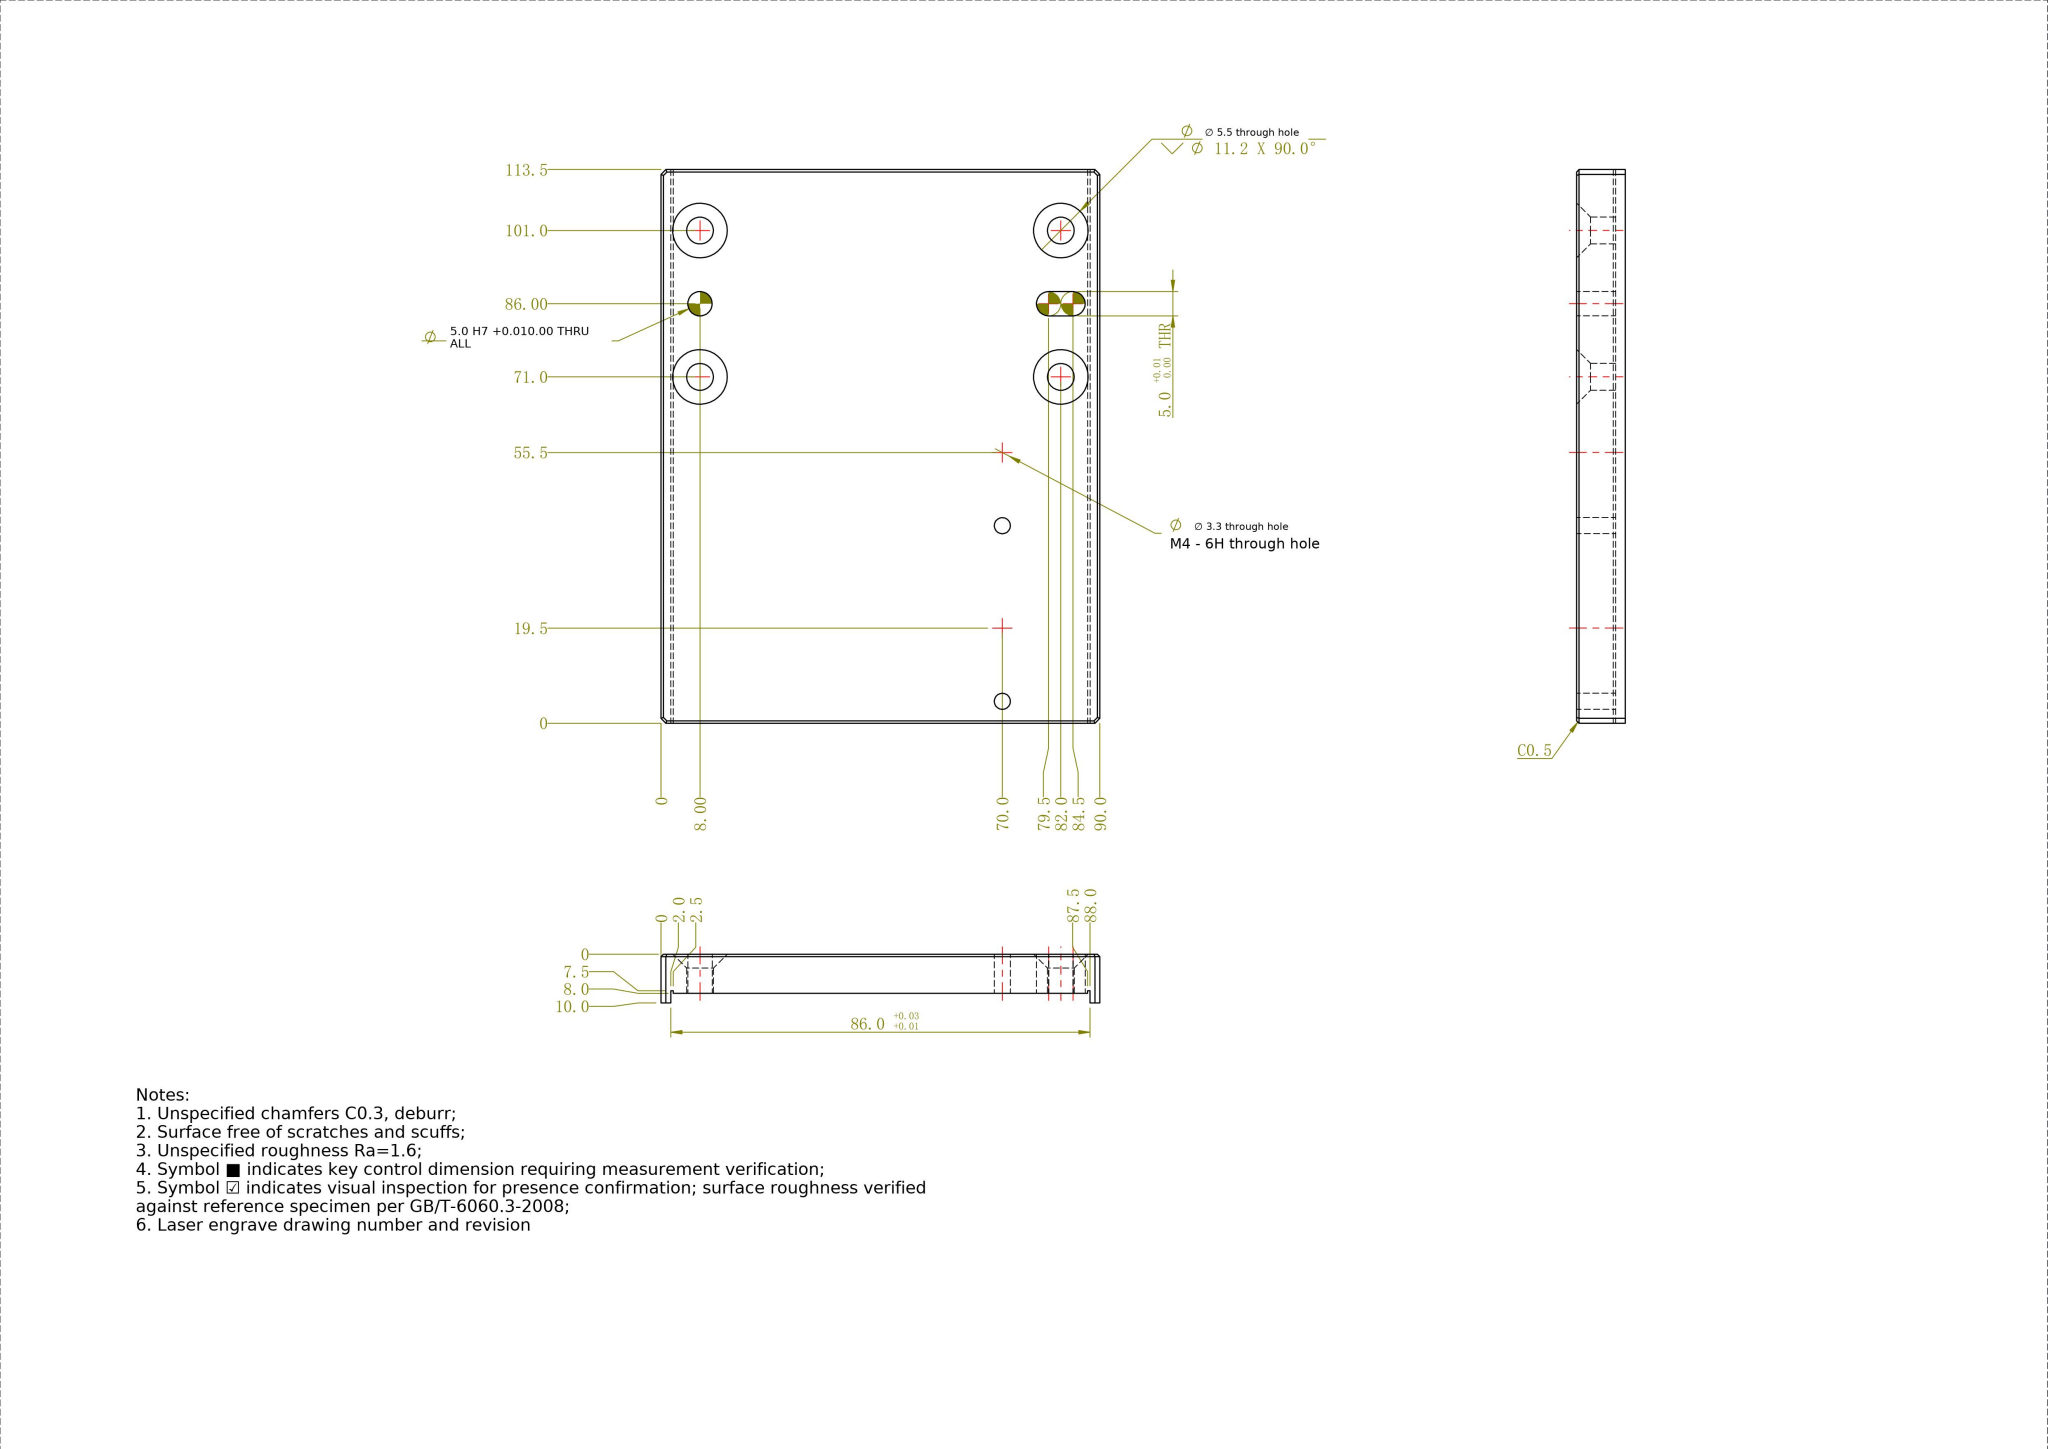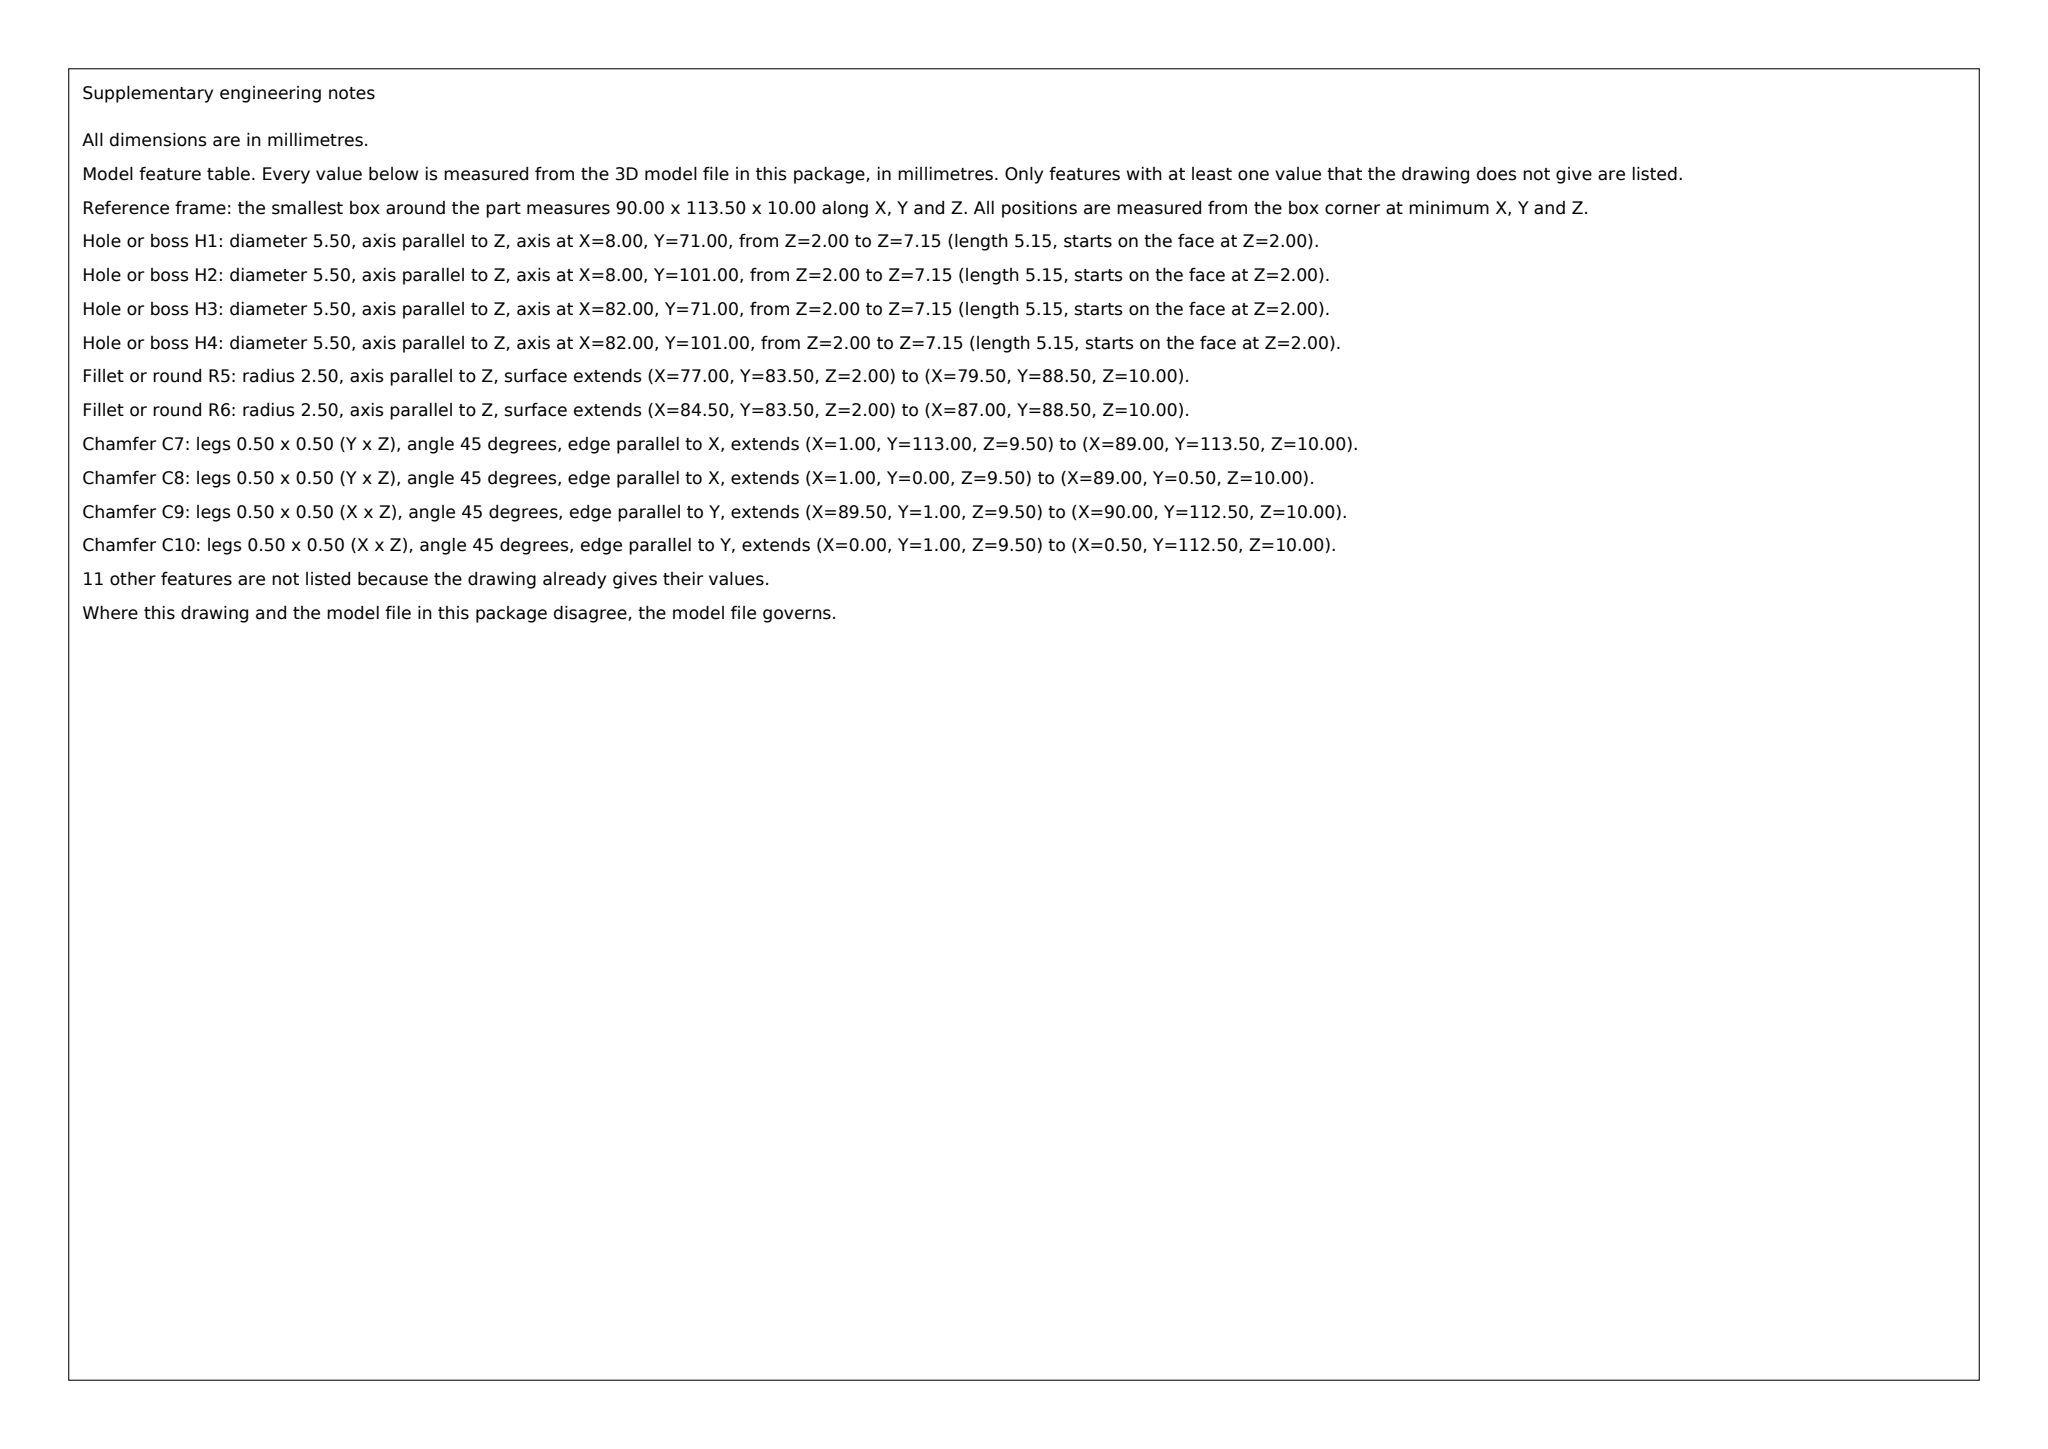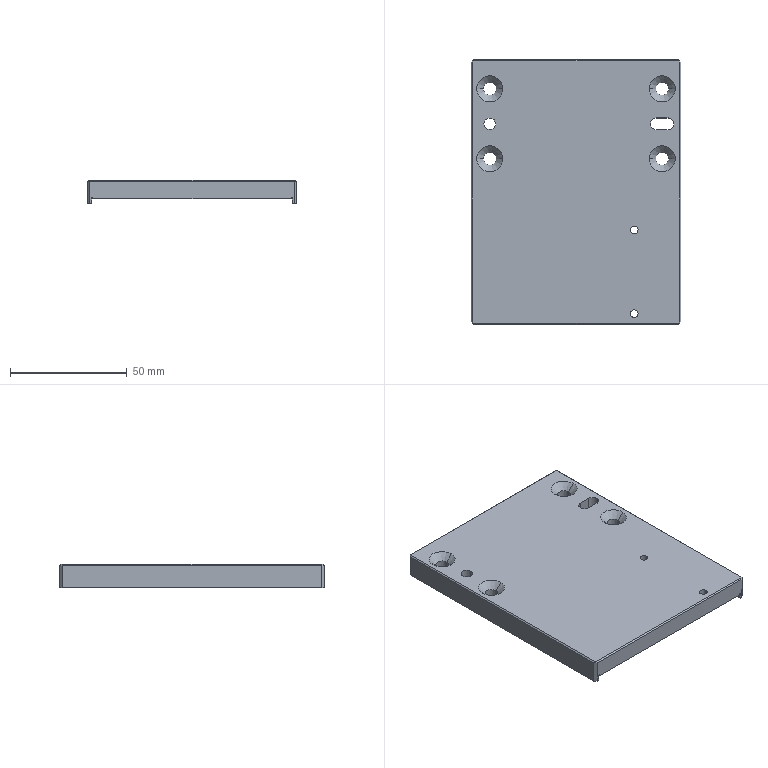Part | SolidWorks | mm | 1 solid | 53 faces | box 90 x 113.5 x 10 mm | volume 80712 mm3 | plane 28 | cylinder 17 | cone 8 | commonest cylinder face diameters 5.5 x8 5 x5 3.3 x4
build123d program:
from build123d import *

# Parameters (mm, degrees)
SKETCH1_W                                            = 90
SKETCH1_H                                            = 113.5
BOSS_EXTRUDE1_DEPTH                                  = 5
SKETCH2_W                                            = 86
SKETCH2_H                                            = 113.5
CUT_EXTRUDE1_DEPTH                                   = 2
SKETCH3_W                                            = 0.5
SKETCH3_H                                            = 0.5
CUT_EXTRUDE2_DEPTH                                   = 126
CHAMFER1_SIZE                                        = 1
CHAMFER2_SIZE                                        = 0.5
COUNTERSUNK_HOLE_1_FOR_M5_HEXAGON_SOCKET_D           = 5.5
COUNTERSUNK_HOLE_1_FOR_M5_HEXAGON_SOCKET_CSINK_D     = 11.2
COUNTERSUNK_HOLE_1_FOR_M5_HEXAGON_SOCKET_CSINK_ANGLE = 90
SIZE_MM_DOWEL_PIN_HOLE_1_D                           = 5
CUT_EXTRUDE3_DEPTH                                   = 126
M4_TAPPED_HOLE1_D                                    = 3.3


with BuildPart() as part:
    # Sketch1 → Boss-Extrude1 (new, symmetric)
    with BuildSketch(Plane.XY):
        Rectangle(SKETCH1_W, SKETCH1_H)
    extrude(amount=BOSS_EXTRUDE1_DEPTH, both=True)

    # Sketch2 → Cut-Extrude1 (cut)
    with BuildSketch(Plane(origin=(0, 0, -5), x_dir=(-1, 0, 0), z_dir=(0, 0, -1))):
        Rectangle(SKETCH2_W, SKETCH2_H)
    extrude(amount=-CUT_EXTRUDE1_DEPTH, mode=Mode.SUBTRACT)

    # Sketch3 → Cut-Extrude2 (cut)
    with BuildSketch(Plane.XZ.offset(56.75)):
        with Locations((-42.75, -2.75)):
            Rectangle(SKETCH3_W, SKETCH3_H)
        with Locations((42.75, -2.75)):
            Rectangle(SKETCH3_W, SKETCH3_H)
    extrude(amount=-CUT_EXTRUDE2_DEPTH, mode=Mode.SUBTRACT)

    # Chamfer1
    chamfer1_edges = [part.edges().sort_by_distance(p)[0] for p in [
        (45, -56.75, 0),
        (-45, -56.75, 0),
        (-45, 56.75, 0),
        (45, 56.75, 0),
    ]]
    chamfer(chamfer1_edges, length=CHAMFER1_SIZE)

    # Chamfer2
    chamfer2_edges = [part.edges().sort_by_distance(p)[0] for p in [
        (45, 0, 5),
        (0, -56.75, 5),
        (0, 56.75, 5),
        (-45, 0, 5),
        (-44.5, -56.25, 5),
        (-44.5, 56.25, 5),
        (44.5, 56.25, 5),
        (44.5, -56.25, 5),
    ]]
    chamfer(chamfer2_edges, length=CHAMFER2_SIZE)

    # Countersunk Hole 1 for M5 Hexagon Socket (through all)
    with Locations(Plane.XY.offset(5)):
        with Locations((-37, 44.25), (37, 44.25), (-37, 14.25), (37, 14.25)):
            CounterSinkHole(COUNTERSUNK_HOLE_1_FOR_M5_HEXAGON_SOCKET_D / 2, COUNTERSUNK_HOLE_1_FOR_M5_HEXAGON_SOCKET_CSINK_D / 2, counter_sink_angle=COUNTERSUNK_HOLE_1_FOR_M5_HEXAGON_SOCKET_CSINK_ANGLE)

    # Size mm Dowel Pin Hole 1 (through all)
    with Locations(Plane.XY.offset(5)):
        with Locations((37, 29.25), (-37, 29.25)):
            Hole(SIZE_MM_DOWEL_PIN_HOLE_1_D / 2)

    # Sketch10 → Cut-Extrude3 (cut)
    with BuildSketch(Plane.XY.offset(5)):
        with BuildLine():
            Line((34.5, 31.75), (39.5, 31.75))
            ThreePointArc((39.5, 31.75), (42, 29.25), (39.5, 26.75))
            Line((39.5, 26.75), (34.5, 26.75))
            ThreePointArc((34.5, 26.75), (32, 29.25), (34.5, 31.75))
        make_face()
    extrude(amount=-CUT_EXTRUDE3_DEPTH, mode=Mode.SUBTRACT)

    # M4 Tapped Hole1 (through all)
    with Locations(Plane.XY.offset(5)):
        with Locations((25, -52.25), (25, -16.25)):
            Hole(M4_TAPPED_HOLE1_D / 2)


solid = part.part